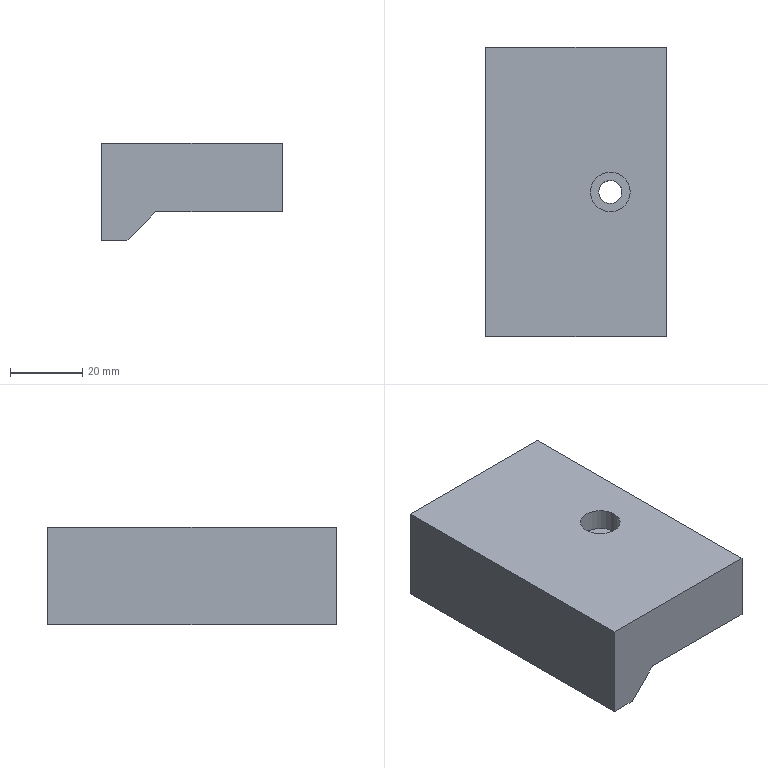Component | NX | 1 | 1 solid | 11 faces | box 50 x 80 x 27 mm | volume 82052 mm3 | plane 9 | cylinder 2 | commonest cylinder face diameters 6.4 x1 11 x1
STEP:
#1=CARTESIAN_POINT('',(0.,0.,0.));
#2=DIRECTION('',(0.,0.,1.));
#3=DIRECTION('',(1.,0.,0.));
#4=AXIS2_PLACEMENT_3D('',#1,#2,#3);
#5=CARTESIAN_POINT('',(-96.,40.,179.));
#6=VERTEX_POINT('',#5);
#7=CARTESIAN_POINT('',(-89.,40.,179.));
#8=VERTEX_POINT('',#7);
#9=CARTESIAN_POINT('',(-96.,40.,179.));
#10=DIRECTION('',(1.,0.,0.));
#11=VECTOR('',#10,1.);
#12=LINE('',#9,#11);
#13=CARTESIAN_POINT('',(-96.,-40.,179.));
#14=DIRECTION('',(0.,0.,1.));
#15=DIRECTION('',(0.,-1.,0.));
#16=AXIS2_PLACEMENT_3D('',#13,#14,#15);
#17=PLANE('',#16);
#18=CARTESIAN_POINT('',(-80.,0.));
#19=DIRECTION('',(0.,1.));
#20=VECTOR('',#19,1.);
#21=LINE('',#18,#20);
#22=(GEOMETRIC_REPRESENTATION_CONTEXT(2)PARAMETRIC_REPRESENTATION_CONTEXT()REPRESENTATION_CONTEXT('',''));
#23=DEFINITIONAL_REPRESENTATION('',(#21),#22);
#24=PCURVE('',#17,#23);
#25=CARTESIAN_POINT('',(-96.,40.,187.));
#26=DIRECTION('',(0.,-1.,0.));
#27=DIRECTION('',(0.,0.,-1.));
#28=AXIS2_PLACEMENT_3D('',#25,#26,#27);
#29=PLANE('',#28);
#30=CARTESIAN_POINT('',(8.,0.));
#31=DIRECTION('',(0.,1.));
#32=VECTOR('',#31,1.);
#33=LINE('',#30,#32);
#34=(GEOMETRIC_REPRESENTATION_CONTEXT(2)PARAMETRIC_REPRESENTATION_CONTEXT()REPRESENTATION_CONTEXT('',''));
#35=DEFINITIONAL_REPRESENTATION('',(#33),#34);
#36=PCURVE('',#29,#35);
#37=SURFACE_CURVE('',#12,(#24,#36),.PCURVE_S1.);
#38=EDGE_CURVE('',#6,#8,#37,.T.);
#39=ORIENTED_EDGE('',*,*,#38,.T.);
#40=CARTESIAN_POINT('',(-89.,-40.,179.));
#41=VERTEX_POINT('',#40);
#42=CARTESIAN_POINT('',(-89.,-40.,179.));
#43=DIRECTION('',(0.,1.,0.));
#44=VECTOR('',#43,1.);
#45=LINE('',#42,#44);
#46=CARTESIAN_POINT('',(0.,7.));
#47=DIRECTION('',(-1.,0.));
#48=VECTOR('',#47,1.);
#49=LINE('',#46,#48);
#50=(GEOMETRIC_REPRESENTATION_CONTEXT(2)PARAMETRIC_REPRESENTATION_CONTEXT()REPRESENTATION_CONTEXT('',''));
#51=DEFINITIONAL_REPRESENTATION('',(#49),#50);
#52=PCURVE('',#17,#51);
#53=CARTESIAN_POINT('',(-89.,-40.,179.));
#54=DIRECTION('',(-0.7071,0.,0.7071));
#55=DIRECTION('',(-0.7071,0.,-0.7071));
#56=AXIS2_PLACEMENT_3D('',#53,#54,#55);
#57=PLANE('',#56);
#58=CARTESIAN_POINT('',(0.,0.));
#59=DIRECTION('',(0.,-1.));
#60=VECTOR('',#59,1.);
#61=LINE('',#58,#60);
#62=(GEOMETRIC_REPRESENTATION_CONTEXT(2)PARAMETRIC_REPRESENTATION_CONTEXT()REPRESENTATION_CONTEXT('',''));
#63=DEFINITIONAL_REPRESENTATION('',(#61),#62);
#64=PCURVE('',#57,#63);
#65=SURFACE_CURVE('',#45,(#52,#64),.PCURVE_S1.);
#66=EDGE_CURVE('',#41,#8,#65,.T.);
#67=ORIENTED_EDGE('',*,*,#66,.F.);
#68=CARTESIAN_POINT('',(-96.,-40.,179.));
#69=VERTEX_POINT('',#68);
#70=CARTESIAN_POINT('',(-96.,-40.,179.));
#71=DIRECTION('',(1.,0.,0.));
#72=VECTOR('',#71,1.);
#73=LINE('',#70,#72);
#74=CARTESIAN_POINT('',(0.,0.));
#75=DIRECTION('',(0.,1.));
#76=VECTOR('',#75,1.);
#77=LINE('',#74,#76);
#78=(GEOMETRIC_REPRESENTATION_CONTEXT(2)PARAMETRIC_REPRESENTATION_CONTEXT()REPRESENTATION_CONTEXT('',''));
#79=DEFINITIONAL_REPRESENTATION('',(#77),#78);
#80=PCURVE('',#17,#79);
#81=CARTESIAN_POINT('',(-96.,-40.,187.));
#82=DIRECTION('',(0.,-1.,0.));
#83=DIRECTION('',(0.,0.,-1.));
#84=AXIS2_PLACEMENT_3D('',#81,#82,#83);
#85=PLANE('',#84);
#86=CARTESIAN_POINT('',(8.,0.));
#87=DIRECTION('',(0.,1.));
#88=VECTOR('',#87,1.);
#89=LINE('',#86,#88);
#90=(GEOMETRIC_REPRESENTATION_CONTEXT(2)PARAMETRIC_REPRESENTATION_CONTEXT()REPRESENTATION_CONTEXT('',''));
#91=DEFINITIONAL_REPRESENTATION('',(#89),#90);
#92=PCURVE('',#85,#91);
#93=SURFACE_CURVE('',#73,(#80,#92),.PCURVE_S1.);
#94=EDGE_CURVE('',#69,#41,#93,.T.);
#95=ORIENTED_EDGE('',*,*,#94,.F.);
#96=CARTESIAN_POINT('',(-96.,-40.,179.));
#97=DIRECTION('',(0.,1.,0.));
#98=VECTOR('',#97,1.);
#99=LINE('',#96,#98);
#100=CARTESIAN_POINT('',(0.,0.));
#101=DIRECTION('',(-1.,0.));
#102=VECTOR('',#101,1.);
#103=LINE('',#100,#102);
#104=(GEOMETRIC_REPRESENTATION_CONTEXT(2)PARAMETRIC_REPRESENTATION_CONTEXT()REPRESENTATION_CONTEXT('',''));
#105=DEFINITIONAL_REPRESENTATION('',(#103),#104);
#106=PCURVE('',#17,#105);
#107=CARTESIAN_POINT('',(-96.,-40.,206.));
#108=DIRECTION('',(1.,0.,0.));
#109=DIRECTION('',(-0.,0.,1.));
#110=AXIS2_PLACEMENT_3D('',#107,#108,#109);
#111=PLANE('',#110);
#112=CARTESIAN_POINT('',(-27.,0.));
#113=DIRECTION('',(0.,-1.));
#114=VECTOR('',#113,1.);
#115=LINE('',#112,#114);
#116=(GEOMETRIC_REPRESENTATION_CONTEXT(2)PARAMETRIC_REPRESENTATION_CONTEXT()REPRESENTATION_CONTEXT('',''));
#117=DEFINITIONAL_REPRESENTATION('',(#115),#116);
#118=PCURVE('',#111,#117);
#119=SURFACE_CURVE('',#99,(#106,#118),.PCURVE_S1.);
#120=EDGE_CURVE('',#69,#6,#119,.T.);
#121=ORIENTED_EDGE('',*,*,#120,.T.);
#122=EDGE_LOOP('',(#39,#67,#95,#121));
#123=FACE_BOUND('',#122,.T.);
#124=ADVANCED_FACE('',(#123),#17,.F.);
#125=CARTESIAN_POINT('',(-81.,40.,187.));
#126=VERTEX_POINT('',#125);
#127=CARTESIAN_POINT('',(-89.,40.,179.));
#128=DIRECTION('',(0.7071,0.,0.7071));
#129=VECTOR('',#128,1.);
#130=LINE('',#127,#129);
#131=CARTESIAN_POINT('',(0.,-80.));
#132=DIRECTION('',(-1.,0.));
#133=VECTOR('',#132,1.);
#134=LINE('',#131,#133);
#135=(GEOMETRIC_REPRESENTATION_CONTEXT(2)PARAMETRIC_REPRESENTATION_CONTEXT()REPRESENTATION_CONTEXT('',''));
#136=DEFINITIONAL_REPRESENTATION('',(#134),#135);
#137=PCURVE('',#57,#136);
#138=CARTESIAN_POINT('',(8.,7.));
#139=DIRECTION('',(-0.7071,0.7071));
#140=VECTOR('',#139,1.);
#141=LINE('',#138,#140);
#142=(GEOMETRIC_REPRESENTATION_CONTEXT(2)PARAMETRIC_REPRESENTATION_CONTEXT()REPRESENTATION_CONTEXT('',''));
#143=DEFINITIONAL_REPRESENTATION('',(#141),#142);
#144=PCURVE('',#29,#143);
#145=SURFACE_CURVE('',#130,(#137,#144),.PCURVE_S1.);
#146=EDGE_CURVE('',#8,#126,#145,.T.);
#147=ORIENTED_EDGE('',*,*,#146,.T.);
#148=CARTESIAN_POINT('',(-81.,-40.,187.));
#149=VERTEX_POINT('',#148);
#150=CARTESIAN_POINT('',(-81.,-40.,187.));
#151=DIRECTION('',(0.,1.,0.));
#152=VECTOR('',#151,1.);
#153=LINE('',#150,#152);
#154=CARTESIAN_POINT('',(-11.314,0.));
#155=DIRECTION('',(0.,-1.));
#156=VECTOR('',#155,1.);
#157=LINE('',#154,#156);
#158=(GEOMETRIC_REPRESENTATION_CONTEXT(2)PARAMETRIC_REPRESENTATION_CONTEXT()REPRESENTATION_CONTEXT('',''));
#159=DEFINITIONAL_REPRESENTATION('',(#157),#158);
#160=PCURVE('',#57,#159);
#161=CARTESIAN_POINT('',(-81.,-40.,187.));
#162=DIRECTION('',(0.,0.,1.));
#163=DIRECTION('',(0.,-1.,0.));
#164=AXIS2_PLACEMENT_3D('',#161,#162,#163);
#165=PLANE('',#164);
#166=CARTESIAN_POINT('',(0.,0.));
#167=DIRECTION('',(-1.,0.));
#168=VECTOR('',#167,1.);
#169=LINE('',#166,#168);
#170=(GEOMETRIC_REPRESENTATION_CONTEXT(2)PARAMETRIC_REPRESENTATION_CONTEXT()REPRESENTATION_CONTEXT('',''));
#171=DEFINITIONAL_REPRESENTATION('',(#169),#170);
#172=PCURVE('',#165,#171);
#173=SURFACE_CURVE('',#153,(#160,#172),.PCURVE_S1.);
#174=EDGE_CURVE('',#149,#126,#173,.T.);
#175=ORIENTED_EDGE('',*,*,#174,.F.);
#176=CARTESIAN_POINT('',(-89.,-40.,179.));
#177=DIRECTION('',(0.7071,0.,0.7071));
#178=VECTOR('',#177,1.);
#179=LINE('',#176,#178);
#180=CARTESIAN_POINT('',(0.,0.));
#181=DIRECTION('',(-1.,0.));
#182=VECTOR('',#181,1.);
#183=LINE('',#180,#182);
#184=(GEOMETRIC_REPRESENTATION_CONTEXT(2)PARAMETRIC_REPRESENTATION_CONTEXT()REPRESENTATION_CONTEXT('',''));
#185=DEFINITIONAL_REPRESENTATION('',(#183),#184);
#186=PCURVE('',#57,#185);
#187=CARTESIAN_POINT('',(8.,7.));
#188=DIRECTION('',(-0.7071,0.7071));
#189=VECTOR('',#188,1.);
#190=LINE('',#187,#189);
#191=(GEOMETRIC_REPRESENTATION_CONTEXT(2)PARAMETRIC_REPRESENTATION_CONTEXT()REPRESENTATION_CONTEXT('',''));
#192=DEFINITIONAL_REPRESENTATION('',(#190),#191);
#193=PCURVE('',#85,#192);
#194=SURFACE_CURVE('',#179,(#186,#193),.PCURVE_S1.);
#195=EDGE_CURVE('',#41,#149,#194,.T.);
#196=ORIENTED_EDGE('',*,*,#195,.F.);
#197=ORIENTED_EDGE('',*,*,#66,.T.);
#198=EDGE_LOOP('',(#147,#175,#196,#197));
#199=FACE_BOUND('',#198,.T.);
#200=ADVANCED_FACE('',(#199),#57,.F.);
#201=CARTESIAN_POINT('',(-61.5,-3.2,187.));
#202=VERTEX_POINT('',#201);
#203=CARTESIAN_POINT('',(-58.3,0.,187.));
#204=VERTEX_POINT('',#203);
#205=CARTESIAN_POINT('',(-61.5,0.,187.));
#206=DIRECTION('',(0.,0.,1.));
#207=DIRECTION('',(0.,-1.,0.));
#208=AXIS2_PLACEMENT_3D('',#205,#206,#207);
#209=CIRCLE('',#208,3.2);
#210=CARTESIAN_POINT('',(-40.,19.5));
#211=DIRECTION('',(1.,0.));
#212=AXIS2_PLACEMENT_2D('',#210,#211);
#213=CIRCLE('',#212,3.2);
#214=(GEOMETRIC_REPRESENTATION_CONTEXT(2)PARAMETRIC_REPRESENTATION_CONTEXT()REPRESENTATION_CONTEXT('',''));
#215=DEFINITIONAL_REPRESENTATION('',(#213),#214);
#216=PCURVE('',#165,#215);
#217=CARTESIAN_POINT('',(-61.5,0.,156.));
#218=DIRECTION('',(0.,0.,-1.));
#219=DIRECTION('',(1.,0.,0.));
#220=AXIS2_PLACEMENT_3D('',#217,#218,#219);
#221=CYLINDRICAL_SURFACE('',#220,3.2);
#222=CARTESIAN_POINT('',(1.571,-31.));
#223=DIRECTION('',(-1.,0.));
#224=VECTOR('',#223,1.);
#225=LINE('',#222,#224);
#226=(GEOMETRIC_REPRESENTATION_CONTEXT(2)PARAMETRIC_REPRESENTATION_CONTEXT()REPRESENTATION_CONTEXT('',''));
#227=DEFINITIONAL_REPRESENTATION('',(#225),#226);
#228=PCURVE('',#221,#227);
#229=SURFACE_CURVE('',#209,(#216,#228),.PCURVE_S1.);
#230=EDGE_CURVE('',#202,#204,#229,.T.);
#231=ORIENTED_EDGE('',*,*,#230,.T.);
#232=CARTESIAN_POINT('',(-61.5,0.,187.));
#233=DIRECTION('',(0.,0.,1.));
#234=DIRECTION('',(0.,-1.,0.));
#235=AXIS2_PLACEMENT_3D('',#232,#233,#234);
#236=CIRCLE('',#235,3.2);
#237=CARTESIAN_POINT('',(-40.,19.5));
#238=DIRECTION('',(1.,0.));
#239=AXIS2_PLACEMENT_2D('',#237,#238);
#240=CIRCLE('',#239,3.2);
#241=(GEOMETRIC_REPRESENTATION_CONTEXT(2)PARAMETRIC_REPRESENTATION_CONTEXT()REPRESENTATION_CONTEXT('',''));
#242=DEFINITIONAL_REPRESENTATION('',(#240),#241);
#243=PCURVE('',#165,#242);
#244=CARTESIAN_POINT('',(7.854,-31.));
#245=DIRECTION('',(-1.,0.));
#246=VECTOR('',#245,1.);
#247=LINE('',#244,#246);
#248=(GEOMETRIC_REPRESENTATION_CONTEXT(2)PARAMETRIC_REPRESENTATION_CONTEXT()REPRESENTATION_CONTEXT('',''));
#249=DEFINITIONAL_REPRESENTATION('',(#247),#248);
#250=PCURVE('',#221,#249);
#251=SURFACE_CURVE('',#236,(#243,#250),.PCURVE_S1.);
#252=EDGE_CURVE('',#204,#202,#251,.T.);
#253=ORIENTED_EDGE('',*,*,#252,.T.);
#254=EDGE_LOOP('',(#231,#253));
#255=FACE_BOUND('',#254,.T.);
#256=CARTESIAN_POINT('',(-46.,40.,187.));
#257=VERTEX_POINT('',#256);
#258=CARTESIAN_POINT('',(-81.,40.,187.));
#259=DIRECTION('',(1.,0.,0.));
#260=VECTOR('',#259,1.);
#261=LINE('',#258,#260);
#262=CARTESIAN_POINT('',(-80.,0.));
#263=DIRECTION('',(0.,1.));
#264=VECTOR('',#263,1.);
#265=LINE('',#262,#264);
#266=(GEOMETRIC_REPRESENTATION_CONTEXT(2)PARAMETRIC_REPRESENTATION_CONTEXT()REPRESENTATION_CONTEXT('',''));
#267=DEFINITIONAL_REPRESENTATION('',(#265),#266);
#268=PCURVE('',#165,#267);
#269=CARTESIAN_POINT('',(0.,15.));
#270=DIRECTION('',(0.,1.));
#271=VECTOR('',#270,1.);
#272=LINE('',#269,#271);
#273=(GEOMETRIC_REPRESENTATION_CONTEXT(2)PARAMETRIC_REPRESENTATION_CONTEXT()REPRESENTATION_CONTEXT('',''));
#274=DEFINITIONAL_REPRESENTATION('',(#272),#273);
#275=PCURVE('',#29,#274);
#276=SURFACE_CURVE('',#261,(#268,#275),.PCURVE_S1.);
#277=EDGE_CURVE('',#126,#257,#276,.T.);
#278=ORIENTED_EDGE('',*,*,#277,.T.);
#279=CARTESIAN_POINT('',(-46.,-40.,187.));
#280=VERTEX_POINT('',#279);
#281=CARTESIAN_POINT('',(-46.,-40.,187.));
#282=DIRECTION('',(0.,1.,0.));
#283=VECTOR('',#282,1.);
#284=LINE('',#281,#283);
#285=CARTESIAN_POINT('',(0.,35.));
#286=DIRECTION('',(-1.,0.));
#287=VECTOR('',#286,1.);
#288=LINE('',#285,#287);
#289=(GEOMETRIC_REPRESENTATION_CONTEXT(2)PARAMETRIC_REPRESENTATION_CONTEXT()REPRESENTATION_CONTEXT('',''));
#290=DEFINITIONAL_REPRESENTATION('',(#288),#289);
#291=PCURVE('',#165,#290);
#292=CARTESIAN_POINT('',(-46.,-40.,187.));
#293=DIRECTION('',(-1.,0.,0.));
#294=DIRECTION('',(0.,0.,-1.));
#295=AXIS2_PLACEMENT_3D('',#292,#293,#294);
#296=PLANE('',#295);
#297=CARTESIAN_POINT('',(0.,0.));
#298=DIRECTION('',(0.,-1.));
#299=VECTOR('',#298,1.);
#300=LINE('',#297,#299);
#301=(GEOMETRIC_REPRESENTATION_CONTEXT(2)PARAMETRIC_REPRESENTATION_CONTEXT()REPRESENTATION_CONTEXT('',''));
#302=DEFINITIONAL_REPRESENTATION('',(#300),#301);
#303=PCURVE('',#296,#302);
#304=SURFACE_CURVE('',#284,(#291,#303),.PCURVE_S1.);
#305=EDGE_CURVE('',#280,#257,#304,.T.);
#306=ORIENTED_EDGE('',*,*,#305,.F.);
#307=CARTESIAN_POINT('',(-81.,-40.,187.));
#308=DIRECTION('',(1.,0.,0.));
#309=VECTOR('',#308,1.);
#310=LINE('',#307,#309);
#311=CARTESIAN_POINT('',(0.,0.));
#312=DIRECTION('',(0.,1.));
#313=VECTOR('',#312,1.);
#314=LINE('',#311,#313);
#315=(GEOMETRIC_REPRESENTATION_CONTEXT(2)PARAMETRIC_REPRESENTATION_CONTEXT()REPRESENTATION_CONTEXT('',''));
#316=DEFINITIONAL_REPRESENTATION('',(#314),#315);
#317=PCURVE('',#165,#316);
#318=CARTESIAN_POINT('',(0.,15.));
#319=DIRECTION('',(0.,1.));
#320=VECTOR('',#319,1.);
#321=LINE('',#318,#320);
#322=(GEOMETRIC_REPRESENTATION_CONTEXT(2)PARAMETRIC_REPRESENTATION_CONTEXT()REPRESENTATION_CONTEXT('',''));
#323=DEFINITIONAL_REPRESENTATION('',(#321),#322);
#324=PCURVE('',#85,#323);
#325=SURFACE_CURVE('',#310,(#317,#324),.PCURVE_S1.);
#326=EDGE_CURVE('',#149,#280,#325,.T.);
#327=ORIENTED_EDGE('',*,*,#326,.F.);
#328=ORIENTED_EDGE('',*,*,#174,.T.);
#329=EDGE_LOOP('',(#278,#306,#327,#328));
#330=FACE_BOUND('',#329,.T.);
#331=ADVANCED_FACE('',(#255,#330),#165,.F.);
#332=CARTESIAN_POINT('',(-46.,40.,206.));
#333=VERTEX_POINT('',#332);
#334=CARTESIAN_POINT('',(-46.,40.,187.));
#335=DIRECTION('',(0.,0.,1.));
#336=VECTOR('',#335,1.);
#337=LINE('',#334,#336);
#338=CARTESIAN_POINT('',(0.,-80.));
#339=DIRECTION('',(-1.,0.));
#340=VECTOR('',#339,1.);
#341=LINE('',#338,#340);
#342=(GEOMETRIC_REPRESENTATION_CONTEXT(2)PARAMETRIC_REPRESENTATION_CONTEXT()REPRESENTATION_CONTEXT('',''));
#343=DEFINITIONAL_REPRESENTATION('',(#341),#342);
#344=PCURVE('',#296,#343);
#345=CARTESIAN_POINT('',(0.,50.));
#346=DIRECTION('',(-1.,0.));
#347=VECTOR('',#346,1.);
#348=LINE('',#345,#347);
#349=(GEOMETRIC_REPRESENTATION_CONTEXT(2)PARAMETRIC_REPRESENTATION_CONTEXT()REPRESENTATION_CONTEXT('',''));
#350=DEFINITIONAL_REPRESENTATION('',(#348),#349);
#351=PCURVE('',#29,#350);
#352=SURFACE_CURVE('',#337,(#344,#351),.PCURVE_S1.);
#353=EDGE_CURVE('',#257,#333,#352,.T.);
#354=ORIENTED_EDGE('',*,*,#353,.T.);
#355=CARTESIAN_POINT('',(-46.,-40.,206.));
#356=VERTEX_POINT('',#355);
#357=CARTESIAN_POINT('',(-46.,-40.,206.));
#358=DIRECTION('',(0.,1.,0.));
#359=VECTOR('',#358,1.);
#360=LINE('',#357,#359);
#361=CARTESIAN_POINT('',(-19.,0.));
#362=DIRECTION('',(0.,-1.));
#363=VECTOR('',#362,1.);
#364=LINE('',#361,#363);
#365=(GEOMETRIC_REPRESENTATION_CONTEXT(2)PARAMETRIC_REPRESENTATION_CONTEXT()REPRESENTATION_CONTEXT('',''));
#366=DEFINITIONAL_REPRESENTATION('',(#364),#365);
#367=PCURVE('',#296,#366);
#368=CARTESIAN_POINT('',(-46.,-40.,206.));
#369=DIRECTION('',(0.,0.,-1.));
#370=DIRECTION('',(1.,0.,0.));
#371=AXIS2_PLACEMENT_3D('',#368,#369,#370);
#372=PLANE('',#371);
#373=CARTESIAN_POINT('',(0.,0.));
#374=DIRECTION('',(0.,-1.));
#375=VECTOR('',#374,1.);
#376=LINE('',#373,#375);
#377=(GEOMETRIC_REPRESENTATION_CONTEXT(2)PARAMETRIC_REPRESENTATION_CONTEXT()REPRESENTATION_CONTEXT('',''));
#378=DEFINITIONAL_REPRESENTATION('',(#376),#377);
#379=PCURVE('',#372,#378);
#380=SURFACE_CURVE('',#360,(#367,#379),.PCURVE_S1.);
#381=EDGE_CURVE('',#356,#333,#380,.T.);
#382=ORIENTED_EDGE('',*,*,#381,.F.);
#383=CARTESIAN_POINT('',(-46.,-40.,187.));
#384=DIRECTION('',(0.,0.,1.));
#385=VECTOR('',#384,1.);
#386=LINE('',#383,#385);
#387=CARTESIAN_POINT('',(0.,0.));
#388=DIRECTION('',(-1.,0.));
#389=VECTOR('',#388,1.);
#390=LINE('',#387,#389);
#391=(GEOMETRIC_REPRESENTATION_CONTEXT(2)PARAMETRIC_REPRESENTATION_CONTEXT()REPRESENTATION_CONTEXT('',''));
#392=DEFINITIONAL_REPRESENTATION('',(#390),#391);
#393=PCURVE('',#296,#392);
#394=CARTESIAN_POINT('',(0.,50.));
#395=DIRECTION('',(-1.,0.));
#396=VECTOR('',#395,1.);
#397=LINE('',#394,#396);
#398=(GEOMETRIC_REPRESENTATION_CONTEXT(2)PARAMETRIC_REPRESENTATION_CONTEXT()REPRESENTATION_CONTEXT('',''));
#399=DEFINITIONAL_REPRESENTATION('',(#397),#398);
#400=PCURVE('',#85,#399);
#401=SURFACE_CURVE('',#386,(#393,#400),.PCURVE_S1.);
#402=EDGE_CURVE('',#280,#356,#401,.T.);
#403=ORIENTED_EDGE('',*,*,#402,.F.);
#404=ORIENTED_EDGE('',*,*,#305,.T.);
#405=EDGE_LOOP('',(#354,#382,#403,#404));
#406=FACE_BOUND('',#405,.T.);
#407=ADVANCED_FACE('',(#406),#296,.F.);
#408=CARTESIAN_POINT('',(-56.,0.,206.));
#409=VERTEX_POINT('',#408);
#410=CARTESIAN_POINT('',(-61.5,0.,206.));
#411=DIRECTION('',(0.,0.,-1.));
#412=DIRECTION('',(1.,0.,0.));
#413=AXIS2_PLACEMENT_3D('',#410,#411,#412);
#414=CIRCLE('',#413,5.5);
#415=CARTESIAN_POINT('',(-15.5,-40.));
#416=DIRECTION('',(1.,0.));
#417=AXIS2_PLACEMENT_2D('',#415,#416);
#418=CIRCLE('',#417,5.5);
#419=(GEOMETRIC_REPRESENTATION_CONTEXT(2)PARAMETRIC_REPRESENTATION_CONTEXT()REPRESENTATION_CONTEXT('',''));
#420=DEFINITIONAL_REPRESENTATION('',(#418),#419);
#421=PCURVE('',#372,#420);
#422=CARTESIAN_POINT('',(-61.5,0.,206.));
#423=DIRECTION('',(0.,0.,-1.));
#424=DIRECTION('',(1.,0.,0.));
#425=AXIS2_PLACEMENT_3D('',#422,#423,#424);
#426=CYLINDRICAL_SURFACE('',#425,5.5);
#427=CARTESIAN_POINT('',(0.,0.));
#428=DIRECTION('',(1.,0.));
#429=VECTOR('',#428,1.);
#430=LINE('',#427,#429);
#431=(GEOMETRIC_REPRESENTATION_CONTEXT(2)PARAMETRIC_REPRESENTATION_CONTEXT()REPRESENTATION_CONTEXT('',''));
#432=DEFINITIONAL_REPRESENTATION('',(#430),#431);
#433=PCURVE('',#426,#432);
#434=SURFACE_CURVE('',#414,(#421,#433),.PCURVE_S1.);
#435=EDGE_CURVE('',#409,#409,#434,.T.);
#436=ORIENTED_EDGE('',*,*,#435,.T.);
#437=EDGE_LOOP('',(#436));
#438=FACE_BOUND('',#437,.T.);
#439=CARTESIAN_POINT('',(-96.,40.,206.));
#440=VERTEX_POINT('',#439);
#441=CARTESIAN_POINT('',(-46.,40.,206.));
#442=DIRECTION('',(-1.,0.,-0.));
#443=VECTOR('',#442,1.);
#444=LINE('',#441,#443);
#445=CARTESIAN_POINT('',(0.,-80.));
#446=DIRECTION('',(-1.,0.));
#447=VECTOR('',#446,1.);
#448=LINE('',#445,#447);
#449=(GEOMETRIC_REPRESENTATION_CONTEXT(2)PARAMETRIC_REPRESENTATION_CONTEXT()REPRESENTATION_CONTEXT('',''));
#450=DEFINITIONAL_REPRESENTATION('',(#448),#449);
#451=PCURVE('',#372,#450);
#452=CARTESIAN_POINT('',(-19.,50.));
#453=DIRECTION('',(0.,-1.));
#454=VECTOR('',#453,1.);
#455=LINE('',#452,#454);
#456=(GEOMETRIC_REPRESENTATION_CONTEXT(2)PARAMETRIC_REPRESENTATION_CONTEXT()REPRESENTATION_CONTEXT('',''));
#457=DEFINITIONAL_REPRESENTATION('',(#455),#456);
#458=PCURVE('',#29,#457);
#459=SURFACE_CURVE('',#444,(#451,#458),.PCURVE_S1.);
#460=EDGE_CURVE('',#333,#440,#459,.T.);
#461=ORIENTED_EDGE('',*,*,#460,.T.);
#462=CARTESIAN_POINT('',(-96.,-40.,206.));
#463=VERTEX_POINT('',#462);
#464=CARTESIAN_POINT('',(-96.,-40.,206.));
#465=DIRECTION('',(0.,1.,0.));
#466=VECTOR('',#465,1.);
#467=LINE('',#464,#466);
#468=CARTESIAN_POINT('',(-50.,0.));
#469=DIRECTION('',(0.,-1.));
#470=VECTOR('',#469,1.);
#471=LINE('',#468,#470);
#472=(GEOMETRIC_REPRESENTATION_CONTEXT(2)PARAMETRIC_REPRESENTATION_CONTEXT()REPRESENTATION_CONTEXT('',''));
#473=DEFINITIONAL_REPRESENTATION('',(#471),#472);
#474=PCURVE('',#372,#473);
#475=CARTESIAN_POINT('',(0.,0.));
#476=DIRECTION('',(0.,-1.));
#477=VECTOR('',#476,1.);
#478=LINE('',#475,#477);
#479=(GEOMETRIC_REPRESENTATION_CONTEXT(2)PARAMETRIC_REPRESENTATION_CONTEXT()REPRESENTATION_CONTEXT('',''));
#480=DEFINITIONAL_REPRESENTATION('',(#478),#479);
#481=PCURVE('',#111,#480);
#482=SURFACE_CURVE('',#467,(#474,#481),.PCURVE_S1.);
#483=EDGE_CURVE('',#463,#440,#482,.T.);
#484=ORIENTED_EDGE('',*,*,#483,.F.);
#485=CARTESIAN_POINT('',(-46.,-40.,206.));
#486=DIRECTION('',(-1.,0.,-0.));
#487=VECTOR('',#486,1.);
#488=LINE('',#485,#487);
#489=CARTESIAN_POINT('',(0.,0.));
#490=DIRECTION('',(-1.,0.));
#491=VECTOR('',#490,1.);
#492=LINE('',#489,#491);
#493=(GEOMETRIC_REPRESENTATION_CONTEXT(2)PARAMETRIC_REPRESENTATION_CONTEXT()REPRESENTATION_CONTEXT('',''));
#494=DEFINITIONAL_REPRESENTATION('',(#492),#493);
#495=PCURVE('',#372,#494);
#496=CARTESIAN_POINT('',(-19.,50.));
#497=DIRECTION('',(0.,-1.));
#498=VECTOR('',#497,1.);
#499=LINE('',#496,#498);
#500=(GEOMETRIC_REPRESENTATION_CONTEXT(2)PARAMETRIC_REPRESENTATION_CONTEXT()REPRESENTATION_CONTEXT('',''));
#501=DEFINITIONAL_REPRESENTATION('',(#499),#500);
#502=PCURVE('',#85,#501);
#503=SURFACE_CURVE('',#488,(#495,#502),.PCURVE_S1.);
#504=EDGE_CURVE('',#356,#463,#503,.T.);
#505=ORIENTED_EDGE('',*,*,#504,.F.);
#506=ORIENTED_EDGE('',*,*,#381,.T.);
#507=EDGE_LOOP('',(#461,#484,#505,#506));
#508=FACE_BOUND('',#507,.T.);
#509=ADVANCED_FACE('',(#438,#508),#372,.F.);
#510=CARTESIAN_POINT('',(-96.,40.,206.));
#511=DIRECTION('',(0.,0.,-1.));
#512=VECTOR('',#511,1.);
#513=LINE('',#510,#512);
#514=CARTESIAN_POINT('',(0.,-80.));
#515=DIRECTION('',(-1.,0.));
#516=VECTOR('',#515,1.);
#517=LINE('',#514,#516);
#518=(GEOMETRIC_REPRESENTATION_CONTEXT(2)PARAMETRIC_REPRESENTATION_CONTEXT()REPRESENTATION_CONTEXT('',''));
#519=DEFINITIONAL_REPRESENTATION('',(#517),#518);
#520=PCURVE('',#111,#519);
#521=CARTESIAN_POINT('',(-19.,0.));
#522=DIRECTION('',(1.,0.));
#523=VECTOR('',#522,1.);
#524=LINE('',#521,#523);
#525=(GEOMETRIC_REPRESENTATION_CONTEXT(2)PARAMETRIC_REPRESENTATION_CONTEXT()REPRESENTATION_CONTEXT('',''));
#526=DEFINITIONAL_REPRESENTATION('',(#524),#525);
#527=PCURVE('',#29,#526);
#528=SURFACE_CURVE('',#513,(#520,#527),.PCURVE_S1.);
#529=EDGE_CURVE('',#440,#6,#528,.T.);
#530=ORIENTED_EDGE('',*,*,#529,.T.);
#531=ORIENTED_EDGE('',*,*,#120,.F.);
#532=CARTESIAN_POINT('',(-96.,-40.,187.));
#533=DIRECTION('',(0.,0.,-1.));
#534=VECTOR('',#533,1.);
#535=LINE('',#532,#534);
#536=CARTESIAN_POINT('',(-19.,0.));
#537=DIRECTION('',(-1.,0.));
#538=VECTOR('',#537,1.);
#539=LINE('',#536,#538);
#540=(GEOMETRIC_REPRESENTATION_CONTEXT(2)PARAMETRIC_REPRESENTATION_CONTEXT()REPRESENTATION_CONTEXT('',''));
#541=DEFINITIONAL_REPRESENTATION('',(#539),#540);
#542=PCURVE('',#111,#541);
#543=CARTESIAN_POINT('',(0.,0.));
#544=DIRECTION('',(1.,0.));
#545=VECTOR('',#544,1.);
#546=LINE('',#543,#545);
#547=(GEOMETRIC_REPRESENTATION_CONTEXT(2)PARAMETRIC_REPRESENTATION_CONTEXT()REPRESENTATION_CONTEXT('',''));
#548=DEFINITIONAL_REPRESENTATION('',(#546),#547);
#549=PCURVE('',#85,#548);
#550=SURFACE_CURVE('',#535,(#542,#549),.PCURVE_S1.);
#551=EDGE_CURVE('',#463,#69,#550,.T.);
#552=ORIENTED_EDGE('',*,*,#551,.F.);
#553=ORIENTED_EDGE('',*,*,#483,.T.);
#554=EDGE_LOOP('',(#530,#531,#552,#553));
#555=FACE_BOUND('',#554,.T.);
#556=ADVANCED_FACE('',(#555),#111,.F.);
#557=ORIENTED_EDGE('',*,*,#551,.T.);
#558=ORIENTED_EDGE('',*,*,#94,.T.);
#559=ORIENTED_EDGE('',*,*,#195,.T.);
#560=ORIENTED_EDGE('',*,*,#326,.T.);
#561=ORIENTED_EDGE('',*,*,#402,.T.);
#562=ORIENTED_EDGE('',*,*,#504,.T.);
#563=EDGE_LOOP('',(#557,#558,#559,#560,#561,#562));
#564=FACE_BOUND('',#563,.T.);
#565=ADVANCED_FACE('',(#564),#85,.T.);
#566=ORIENTED_EDGE('',*,*,#38,.F.);
#567=ORIENTED_EDGE('',*,*,#529,.F.);
#568=ORIENTED_EDGE('',*,*,#460,.F.);
#569=ORIENTED_EDGE('',*,*,#353,.F.);
#570=ORIENTED_EDGE('',*,*,#277,.F.);
#571=ORIENTED_EDGE('',*,*,#146,.F.);
#572=EDGE_LOOP('',(#566,#567,#568,#569,#570,#571));
#573=FACE_BOUND('',#572,.T.);
#574=ADVANCED_FACE('',(#573),#29,.F.);
#575=CARTESIAN_POINT('',(-58.3,0.,200.));
#576=VERTEX_POINT('',#575);
#577=CARTESIAN_POINT('',(-61.5,0.,200.));
#578=DIRECTION('',(-0.,0.,1.));
#579=DIRECTION('',(1.,0.,0.));
#580=AXIS2_PLACEMENT_3D('',#577,#578,#579);
#581=CIRCLE('',#580,3.2);
#582=CARTESIAN_POINT('',(6.283,-44.));
#583=DIRECTION('',(-1.,0.));
#584=VECTOR('',#583,1.);
#585=LINE('',#582,#584);
#586=(GEOMETRIC_REPRESENTATION_CONTEXT(2)PARAMETRIC_REPRESENTATION_CONTEXT()REPRESENTATION_CONTEXT('',''));
#587=DEFINITIONAL_REPRESENTATION('',(#585),#586);
#588=PCURVE('',#221,#587);
#589=CARTESIAN_POINT('',(-61.5,0.,200.));
#590=DIRECTION('',(0.,0.,-1.));
#591=DIRECTION('',(1.,0.,0.));
#592=AXIS2_PLACEMENT_3D('',#589,#590,#591);
#593=PLANE('',#592);
#594=CARTESIAN_POINT('',(3.2,0.));
#595=CARTESIAN_POINT('',(3.2,-5.543));
#596=CARTESIAN_POINT('',(-1.6,-2.771));
#597=CARTESIAN_POINT('',(-6.4,-0.));
#598=CARTESIAN_POINT('',(-1.6,2.771));
#599=CARTESIAN_POINT('',(3.2,5.543));
#600=CARTESIAN_POINT('',(3.2,0.));
#601=(BOUNDED_CURVE()B_SPLINE_CURVE(2,(#594,#595,#596,#597,#598,#599,#600),.UNSPECIFIED.,.T.,.F.)B_SPLINE_CURVE_WITH_KNOTS((1,2,2,2,2,1),(-2.094,0.,2.094,4.189,6.283,8.378),.UNSPECIFIED.)CURVE()GEOMETRIC_REPRESENTATION_ITEM()RATIONAL_B_SPLINE_CURVE((1.,0.5,1.,0.5,1.,0.5,1.))REPRESENTATION_ITEM(''));
#602=(GEOMETRIC_REPRESENTATION_CONTEXT(2)PARAMETRIC_REPRESENTATION_CONTEXT()REPRESENTATION_CONTEXT('',''));
#603=DEFINITIONAL_REPRESENTATION('',(#601),#602);
#604=PCURVE('',#593,#603);
#605=SURFACE_CURVE('',#581,(#588,#604),.PCURVE_S1.);
#606=EDGE_CURVE('',#576,#576,#605,.T.);
#607=ORIENTED_EDGE('',*,*,#606,.F.);
#608=CARTESIAN_POINT('',(-58.3,0.,200.));
#609=CARTESIAN_POINT('',(-58.3,0.,187.));
#610=B_SPLINE_CURVE_WITH_KNOTS('',1,(#608,#609),.UNSPECIFIED.,.F.,.F.,(2,2),(-44.,-31.),.PIECEWISE_BEZIER_KNOTS.);
#611=CARTESIAN_POINT('',(6.283,0.));
#612=DIRECTION('',(0.,1.));
#613=VECTOR('',#612,1.);
#614=LINE('',#611,#613);
#615=(GEOMETRIC_REPRESENTATION_CONTEXT(2)PARAMETRIC_REPRESENTATION_CONTEXT()REPRESENTATION_CONTEXT('',''));
#616=DEFINITIONAL_REPRESENTATION('',(#614),#615);
#617=PCURVE('',#221,#616);
#618=CARTESIAN_POINT('',(0.,0.));
#619=DIRECTION('',(0.,1.));
#620=VECTOR('',#619,1.);
#621=LINE('',#618,#620);
#622=(GEOMETRIC_REPRESENTATION_CONTEXT(2)PARAMETRIC_REPRESENTATION_CONTEXT()REPRESENTATION_CONTEXT('',''));
#623=DEFINITIONAL_REPRESENTATION('',(#621),#622);
#624=PCURVE('',#221,#623);
#625=SEAM_CURVE('',#610,(#617,#624),.PCURVE_S1.);
#626=EDGE_CURVE('',#576,#204,#625,.T.);
#627=ORIENTED_EDGE('',*,*,#626,.T.);
#628=ORIENTED_EDGE('',*,*,#252,.T.);
#629=ORIENTED_EDGE('',*,*,#230,.T.);
#630=ORIENTED_EDGE('',*,*,#626,.F.);
#631=EDGE_LOOP('',(#607,#627,#628,#629,#630));
#632=FACE_BOUND('',#631,.F.);
#633=ADVANCED_FACE('',(#632),#221,.F.);
#634=ORIENTED_EDGE('',*,*,#606,.F.);
#635=EDGE_LOOP('',(#634));
#636=FACE_BOUND('',#635,.T.);
#637=CARTESIAN_POINT('',(-56.,0.,200.));
#638=VERTEX_POINT('',#637);
#639=CARTESIAN_POINT('',(-61.5,0.,200.));
#640=DIRECTION('',(-0.,0.,1.));
#641=DIRECTION('',(1.,0.,0.));
#642=AXIS2_PLACEMENT_3D('',#639,#640,#641);
#643=CIRCLE('',#642,5.5);
#644=CARTESIAN_POINT('',(5.5,0.));
#645=CARTESIAN_POINT('',(5.5,-9.526));
#646=CARTESIAN_POINT('',(-2.75,-4.763));
#647=CARTESIAN_POINT('',(-11.,-0.));
#648=CARTESIAN_POINT('',(-2.75,4.763));
#649=CARTESIAN_POINT('',(5.5,9.526));
#650=CARTESIAN_POINT('',(5.5,0.));
#651=(BOUNDED_CURVE()B_SPLINE_CURVE(2,(#644,#645,#646,#647,#648,#649,#650),.UNSPECIFIED.,.T.,.F.)B_SPLINE_CURVE_WITH_KNOTS((1,2,2,2,2,1),(-2.094,0.,2.094,4.189,6.283,8.378),.UNSPECIFIED.)CURVE()GEOMETRIC_REPRESENTATION_ITEM()RATIONAL_B_SPLINE_CURVE((1.,0.5,1.,0.5,1.,0.5,1.))REPRESENTATION_ITEM(''));
#652=(GEOMETRIC_REPRESENTATION_CONTEXT(2)PARAMETRIC_REPRESENTATION_CONTEXT()REPRESENTATION_CONTEXT('',''));
#653=DEFINITIONAL_REPRESENTATION('',(#651),#652);
#654=PCURVE('',#593,#653);
#655=CARTESIAN_POINT('',(6.283,6.));
#656=DIRECTION('',(-1.,0.));
#657=VECTOR('',#656,1.);
#658=LINE('',#655,#657);
#659=(GEOMETRIC_REPRESENTATION_CONTEXT(2)PARAMETRIC_REPRESENTATION_CONTEXT()REPRESENTATION_CONTEXT('',''));
#660=DEFINITIONAL_REPRESENTATION('',(#658),#659);
#661=PCURVE('',#426,#660);
#662=SURFACE_CURVE('',#643,(#654,#661),.PCURVE_S1.);
#663=EDGE_CURVE('',#638,#638,#662,.T.);
#664=ORIENTED_EDGE('',*,*,#663,.T.);
#665=EDGE_LOOP('',(#664));
#666=FACE_BOUND('',#665,.T.);
#667=ADVANCED_FACE('',(#636,#666),#593,.F.);
#668=ORIENTED_EDGE('',*,*,#663,.T.);
#669=CARTESIAN_POINT('',(-56.,0.,206.));
#670=CARTESIAN_POINT('',(-56.,0.,200.));
#671=B_SPLINE_CURVE_WITH_KNOTS('',1,(#669,#670),.UNSPECIFIED.,.F.,.F.,(2,2),(0.,6.),.PIECEWISE_BEZIER_KNOTS.);
#672=CARTESIAN_POINT('',(0.,0.));
#673=DIRECTION('',(0.,1.));
#674=VECTOR('',#673,1.);
#675=LINE('',#672,#674);
#676=(GEOMETRIC_REPRESENTATION_CONTEXT(2)PARAMETRIC_REPRESENTATION_CONTEXT()REPRESENTATION_CONTEXT('',''));
#677=DEFINITIONAL_REPRESENTATION('',(#675),#676);
#678=PCURVE('',#426,#677);
#679=CARTESIAN_POINT('',(6.283,0.));
#680=DIRECTION('',(0.,1.));
#681=VECTOR('',#680,1.);
#682=LINE('',#679,#681);
#683=(GEOMETRIC_REPRESENTATION_CONTEXT(2)PARAMETRIC_REPRESENTATION_CONTEXT()REPRESENTATION_CONTEXT('',''));
#684=DEFINITIONAL_REPRESENTATION('',(#682),#683);
#685=PCURVE('',#426,#684);
#686=SEAM_CURVE('',#671,(#678,#685),.PCURVE_S1.);
#687=EDGE_CURVE('',#409,#638,#686,.T.);
#688=ORIENTED_EDGE('',*,*,#687,.F.);
#689=ORIENTED_EDGE('',*,*,#435,.T.);
#690=ORIENTED_EDGE('',*,*,#687,.T.);
#691=EDGE_LOOP('',(#668,#688,#689,#690));
#692=FACE_BOUND('',#691,.F.);
#693=ADVANCED_FACE('',(#692),#426,.F.);
#694=CLOSED_SHELL('',(#124,#200,#331,#407,#509,#556,#565,#574,#633,#667,#693));
#695=MANIFOLD_SOLID_BREP('',#694);
#696=(LENGTH_UNIT()NAMED_UNIT(*)SI_UNIT(.MILLI.,.METRE.));
#697=UNCERTAINTY_MEASURE_WITH_UNIT(LENGTH_MEASURE(0.000002),#696,'','');
#698=(NAMED_UNIT(*)PLANE_ANGLE_UNIT()SI_UNIT($,.RADIAN.));
#699=(NAMED_UNIT(*)SI_UNIT($,.STERADIAN.)SOLID_ANGLE_UNIT());
#700=(GEOMETRIC_REPRESENTATION_CONTEXT(3)GLOBAL_UNCERTAINTY_ASSIGNED_CONTEXT((#697))GLOBAL_UNIT_ASSIGNED_CONTEXT((#696,#698,#699))REPRESENTATION_CONTEXT('',''));
#701=ADVANCED_BREP_SHAPE_REPRESENTATION('',(#4,#695),#700);